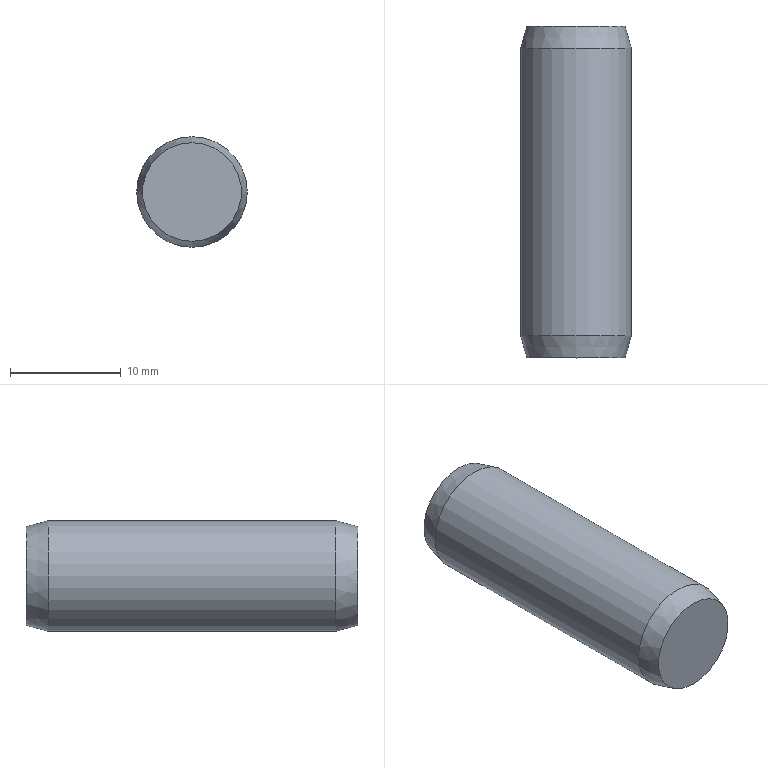Component | NX | GB-T119_1-2000_10X30 | 1 solid | 5 faces | box 10 x 30 x 10 mm | volume 2324 mm3 | plane 2 | cone 2 | cylinder 1 | commonest cylinder face diameters 10 x1
STEP:
#1=CARTESIAN_POINT('',(0.,0.,0.));
#2=DIRECTION('',(0.,0.,1.));
#3=DIRECTION('',(1.,0.,0.));
#4=AXIS2_PLACEMENT_3D('',#1,#2,#3);
#5=CARTESIAN_POINT('',(-40.,80.,-193.464));
#6=VERTEX_POINT('',#5);
#7=CARTESIAN_POINT('',(-40.,80.,-189.));
#8=DIRECTION('',(0.,1.,0.));
#9=DIRECTION('',(0.,0.,-1.));
#10=AXIS2_PLACEMENT_3D('',#7,#8,#9);
#11=CIRCLE('',#10,4.464);
#12=CARTESIAN_POINT('',(-40.,80.,-189.));
#13=DIRECTION('',(0.,1.,0.));
#14=DIRECTION('',(0.,0.,-1.));
#15=AXIS2_PLACEMENT_3D('',#12,#13,#14);
#16=PLANE('',#15);
#17=CARTESIAN_POINT('',(0.,0.));
#18=DIRECTION('',(1.,0.));
#19=AXIS2_PLACEMENT_2D('',#17,#18);
#20=CIRCLE('',#19,4.464);
#21=(GEOMETRIC_REPRESENTATION_CONTEXT(2)PARAMETRIC_REPRESENTATION_CONTEXT()REPRESENTATION_CONTEXT('',''));
#22=DEFINITIONAL_REPRESENTATION('',(#20),#21);
#23=PCURVE('',#16,#22);
#24=CARTESIAN_POINT('',(-40.,80.,-189.));
#25=DIRECTION('',(0.,-1.,0.));
#26=DIRECTION('',(0.,0.,1.));
#27=AXIS2_PLACEMENT_3D('',#24,#25,#26);
#28=CONICAL_SURFACE('',#27,4.464,0.2618);
#29=CARTESIAN_POINT('',(9.425,0.));
#30=DIRECTION('',(-1.,0.));
#31=VECTOR('',#30,1.);
#32=LINE('',#29,#31);
#33=(GEOMETRIC_REPRESENTATION_CONTEXT(2)PARAMETRIC_REPRESENTATION_CONTEXT()REPRESENTATION_CONTEXT('',''));
#34=DEFINITIONAL_REPRESENTATION('',(#32),#33);
#35=PCURVE('',#28,#34);
#36=SURFACE_CURVE('',#11,(#23,#35),.PCURVE_S1.);
#37=EDGE_CURVE('',#6,#6,#36,.T.);
#38=ORIENTED_EDGE('',*,*,#37,.T.);
#39=EDGE_LOOP('',(#38));
#40=FACE_BOUND('',#39,.T.);
#41=ADVANCED_FACE('',(#40),#16,.T.);
#42=CARTESIAN_POINT('',(-40.,78.,-194.));
#43=VERTEX_POINT('',#42);
#44=CARTESIAN_POINT('',(-40.,78.,-189.));
#45=DIRECTION('',(0.,1.,0.));
#46=DIRECTION('',(0.,0.,-1.));
#47=AXIS2_PLACEMENT_3D('',#44,#45,#46);
#48=CIRCLE('',#47,5.);
#49=CARTESIAN_POINT('',(9.425,2.));
#50=DIRECTION('',(-1.,0.));
#51=VECTOR('',#50,1.);
#52=LINE('',#49,#51);
#53=(GEOMETRIC_REPRESENTATION_CONTEXT(2)PARAMETRIC_REPRESENTATION_CONTEXT()REPRESENTATION_CONTEXT('',''));
#54=DEFINITIONAL_REPRESENTATION('',(#52),#53);
#55=PCURVE('',#28,#54);
#56=CARTESIAN_POINT('',(-40.,50.,-189.));
#57=DIRECTION('',(0.,1.,0.));
#58=DIRECTION('',(0.,0.,-1.));
#59=AXIS2_PLACEMENT_3D('',#56,#57,#58);
#60=CYLINDRICAL_SURFACE('',#59,5.);
#61=CARTESIAN_POINT('',(0.,28.));
#62=DIRECTION('',(1.,0.));
#63=VECTOR('',#62,1.);
#64=LINE('',#61,#63);
#65=(GEOMETRIC_REPRESENTATION_CONTEXT(2)PARAMETRIC_REPRESENTATION_CONTEXT()REPRESENTATION_CONTEXT('',''));
#66=DEFINITIONAL_REPRESENTATION('',(#64),#65);
#67=PCURVE('',#60,#66);
#68=SURFACE_CURVE('',#48,(#55,#67),.PCURVE_S1.);
#69=EDGE_CURVE('',#43,#43,#68,.T.);
#70=ORIENTED_EDGE('',*,*,#69,.T.);
#71=CARTESIAN_POINT('',(-40.,80.,-193.464));
#72=CARTESIAN_POINT('',(-40.,78.,-194.));
#73=B_SPLINE_CURVE_WITH_KNOTS('',1,(#71,#72),.UNSPECIFIED.,.F.,.F.,(2,2),(0.,2.071),.PIECEWISE_BEZIER_KNOTS.);
#74=CARTESIAN_POINT('',(3.142,0.));
#75=DIRECTION('',(0.,1.));
#76=VECTOR('',#75,1.);
#77=LINE('',#74,#76);
#78=(GEOMETRIC_REPRESENTATION_CONTEXT(2)PARAMETRIC_REPRESENTATION_CONTEXT()REPRESENTATION_CONTEXT('',''));
#79=DEFINITIONAL_REPRESENTATION('',(#77),#78);
#80=PCURVE('',#28,#79);
#81=CARTESIAN_POINT('',(9.425,0.));
#82=DIRECTION('',(0.,1.));
#83=VECTOR('',#82,1.);
#84=LINE('',#81,#83);
#85=(GEOMETRIC_REPRESENTATION_CONTEXT(2)PARAMETRIC_REPRESENTATION_CONTEXT()REPRESENTATION_CONTEXT('',''));
#86=DEFINITIONAL_REPRESENTATION('',(#84),#85);
#87=PCURVE('',#28,#86);
#88=SEAM_CURVE('',#73,(#80,#87),.PCURVE_S1.);
#89=EDGE_CURVE('',#6,#43,#88,.T.);
#90=ORIENTED_EDGE('',*,*,#89,.F.);
#91=ORIENTED_EDGE('',*,*,#37,.F.);
#92=ORIENTED_EDGE('',*,*,#89,.T.);
#93=EDGE_LOOP('',(#70,#90,#91,#92));
#94=FACE_BOUND('',#93,.T.);
#95=ADVANCED_FACE('',(#94),#28,.T.);
#96=CARTESIAN_POINT('',(-40.,52.,-194.));
#97=VERTEX_POINT('',#96);
#98=CARTESIAN_POINT('',(-40.,52.,-189.));
#99=DIRECTION('',(0.,1.,0.));
#100=DIRECTION('',(0.,0.,-1.));
#101=AXIS2_PLACEMENT_3D('',#98,#99,#100);
#102=CIRCLE('',#101,5.);
#103=CARTESIAN_POINT('',(0.,2.));
#104=DIRECTION('',(1.,0.));
#105=VECTOR('',#104,1.);
#106=LINE('',#103,#105);
#107=(GEOMETRIC_REPRESENTATION_CONTEXT(2)PARAMETRIC_REPRESENTATION_CONTEXT()REPRESENTATION_CONTEXT('',''));
#108=DEFINITIONAL_REPRESENTATION('',(#106),#107);
#109=PCURVE('',#60,#108);
#110=CARTESIAN_POINT('',(-40.,52.,-189.));
#111=DIRECTION('',(0.,1.,0.));
#112=DIRECTION('',(0.,0.,-1.));
#113=AXIS2_PLACEMENT_3D('',#110,#111,#112);
#114=CONICAL_SURFACE('',#113,5.,0.2618);
#115=CARTESIAN_POINT('',(0.,-0.));
#116=DIRECTION('',(1.,0.));
#117=VECTOR('',#116,1.);
#118=LINE('',#115,#117);
#119=(GEOMETRIC_REPRESENTATION_CONTEXT(2)PARAMETRIC_REPRESENTATION_CONTEXT()REPRESENTATION_CONTEXT('',''));
#120=DEFINITIONAL_REPRESENTATION('',(#118),#119);
#121=PCURVE('',#114,#120);
#122=SURFACE_CURVE('',#102,(#109,#121),.PCURVE_S1.);
#123=EDGE_CURVE('',#97,#97,#122,.T.);
#124=ORIENTED_EDGE('',*,*,#123,.T.);
#125=CARTESIAN_POINT('',(-40.,52.,-194.));
#126=CARTESIAN_POINT('',(-40.,78.,-194.));
#127=B_SPLINE_CURVE_WITH_KNOTS('',1,(#125,#126),.UNSPECIFIED.,.F.,.F.,(2,2),(2.,28.),.PIECEWISE_BEZIER_KNOTS.);
#128=CARTESIAN_POINT('',(6.283,0.));
#129=DIRECTION('',(0.,1.));
#130=VECTOR('',#129,1.);
#131=LINE('',#128,#130);
#132=(GEOMETRIC_REPRESENTATION_CONTEXT(2)PARAMETRIC_REPRESENTATION_CONTEXT()REPRESENTATION_CONTEXT('',''));
#133=DEFINITIONAL_REPRESENTATION('',(#131),#132);
#134=PCURVE('',#60,#133);
#135=CARTESIAN_POINT('',(0.,0.));
#136=DIRECTION('',(0.,1.));
#137=VECTOR('',#136,1.);
#138=LINE('',#135,#137);
#139=(GEOMETRIC_REPRESENTATION_CONTEXT(2)PARAMETRIC_REPRESENTATION_CONTEXT()REPRESENTATION_CONTEXT('',''));
#140=DEFINITIONAL_REPRESENTATION('',(#138),#139);
#141=PCURVE('',#60,#140);
#142=SEAM_CURVE('',#127,(#134,#141),.PCURVE_S1.);
#143=EDGE_CURVE('',#97,#43,#142,.T.);
#144=ORIENTED_EDGE('',*,*,#143,.T.);
#145=ORIENTED_EDGE('',*,*,#69,.F.);
#146=ORIENTED_EDGE('',*,*,#143,.F.);
#147=EDGE_LOOP('',(#124,#144,#145,#146));
#148=FACE_BOUND('',#147,.T.);
#149=ADVANCED_FACE('',(#148),#60,.T.);
#150=CARTESIAN_POINT('',(-40.,50.,-193.464));
#151=VERTEX_POINT('',#150);
#152=CARTESIAN_POINT('',(-40.,50.,-189.));
#153=DIRECTION('',(0.,1.,0.));
#154=DIRECTION('',(0.,0.,-1.));
#155=AXIS2_PLACEMENT_3D('',#152,#153,#154);
#156=CIRCLE('',#155,4.464);
#157=CARTESIAN_POINT('',(0.,-2.));
#158=DIRECTION('',(1.,0.));
#159=VECTOR('',#158,1.);
#160=LINE('',#157,#159);
#161=(GEOMETRIC_REPRESENTATION_CONTEXT(2)PARAMETRIC_REPRESENTATION_CONTEXT()REPRESENTATION_CONTEXT('',''));
#162=DEFINITIONAL_REPRESENTATION('',(#160),#161);
#163=PCURVE('',#114,#162);
#164=CARTESIAN_POINT('',(-40.,50.,-184.536));
#165=DIRECTION('',(0.,-1.,0.));
#166=DIRECTION('',(0.,0.,1.));
#167=AXIS2_PLACEMENT_3D('',#164,#165,#166);
#168=PLANE('',#167);
#169=CARTESIAN_POINT('',(-8.928,0.));
#170=CARTESIAN_POINT('',(-8.928,7.732));
#171=CARTESIAN_POINT('',(-2.232,3.866));
#172=CARTESIAN_POINT('',(4.464,0.));
#173=CARTESIAN_POINT('',(-2.232,-3.866));
#174=CARTESIAN_POINT('',(-8.928,-7.732));
#175=CARTESIAN_POINT('',(-8.928,0.));
#176=(BOUNDED_CURVE()B_SPLINE_CURVE(2,(#169,#170,#171,#172,#173,#174,#175),.UNSPECIFIED.,.T.,.F.)B_SPLINE_CURVE_WITH_KNOTS((1,2,2,2,2,1),(-2.094,0.,2.094,4.189,6.283,8.378),.UNSPECIFIED.)CURVE()GEOMETRIC_REPRESENTATION_ITEM()RATIONAL_B_SPLINE_CURVE((1.,0.5,1.,0.5,1.,0.5,1.))REPRESENTATION_ITEM(''));
#177=(GEOMETRIC_REPRESENTATION_CONTEXT(2)PARAMETRIC_REPRESENTATION_CONTEXT()REPRESENTATION_CONTEXT('',''));
#178=DEFINITIONAL_REPRESENTATION('',(#176),#177);
#179=PCURVE('',#168,#178);
#180=SURFACE_CURVE('',#156,(#163,#179),.PCURVE_S1.);
#181=EDGE_CURVE('',#151,#151,#180,.T.);
#182=ORIENTED_EDGE('',*,*,#181,.T.);
#183=CARTESIAN_POINT('',(-40.,50.,-193.464));
#184=CARTESIAN_POINT('',(-40.,52.,-194.));
#185=B_SPLINE_CURVE_WITH_KNOTS('',1,(#183,#184),.UNSPECIFIED.,.F.,.F.,(2,2),(-2.071,-0.),.PIECEWISE_BEZIER_KNOTS.);
#186=CARTESIAN_POINT('',(6.283,0.));
#187=DIRECTION('',(0.,1.));
#188=VECTOR('',#187,1.);
#189=LINE('',#186,#188);
#190=(GEOMETRIC_REPRESENTATION_CONTEXT(2)PARAMETRIC_REPRESENTATION_CONTEXT()REPRESENTATION_CONTEXT('',''));
#191=DEFINITIONAL_REPRESENTATION('',(#189),#190);
#192=PCURVE('',#114,#191);
#193=CARTESIAN_POINT('',(0.,0.));
#194=DIRECTION('',(0.,1.));
#195=VECTOR('',#194,1.);
#196=LINE('',#193,#195);
#197=(GEOMETRIC_REPRESENTATION_CONTEXT(2)PARAMETRIC_REPRESENTATION_CONTEXT()REPRESENTATION_CONTEXT('',''));
#198=DEFINITIONAL_REPRESENTATION('',(#196),#197);
#199=PCURVE('',#114,#198);
#200=SEAM_CURVE('',#185,(#192,#199),.PCURVE_S1.);
#201=EDGE_CURVE('',#151,#97,#200,.T.);
#202=ORIENTED_EDGE('',*,*,#201,.T.);
#203=ORIENTED_EDGE('',*,*,#123,.F.);
#204=ORIENTED_EDGE('',*,*,#201,.F.);
#205=EDGE_LOOP('',(#182,#202,#203,#204));
#206=FACE_BOUND('',#205,.T.);
#207=ADVANCED_FACE('',(#206),#114,.T.);
#208=ORIENTED_EDGE('',*,*,#181,.F.);
#209=EDGE_LOOP('',(#208));
#210=FACE_BOUND('',#209,.T.);
#211=ADVANCED_FACE('',(#210),#168,.T.);
#212=CLOSED_SHELL('',(#41,#95,#149,#207,#211));
#213=MANIFOLD_SOLID_BREP('',#212);
#214=(LENGTH_UNIT()NAMED_UNIT(*)SI_UNIT(.MILLI.,.METRE.));
#215=UNCERTAINTY_MEASURE_WITH_UNIT(LENGTH_MEASURE(0.00001),#214,'','');
#216=(NAMED_UNIT(*)PLANE_ANGLE_UNIT()SI_UNIT($,.RADIAN.));
#217=(NAMED_UNIT(*)SI_UNIT($,.STERADIAN.)SOLID_ANGLE_UNIT());
#218=(GEOMETRIC_REPRESENTATION_CONTEXT(3)GLOBAL_UNCERTAINTY_ASSIGNED_CONTEXT((#215))GLOBAL_UNIT_ASSIGNED_CONTEXT((#214,#216,#217))REPRESENTATION_CONTEXT('',''));
#219=ADVANCED_BREP_SHAPE_REPRESENTATION('',(#4,#213),#218);